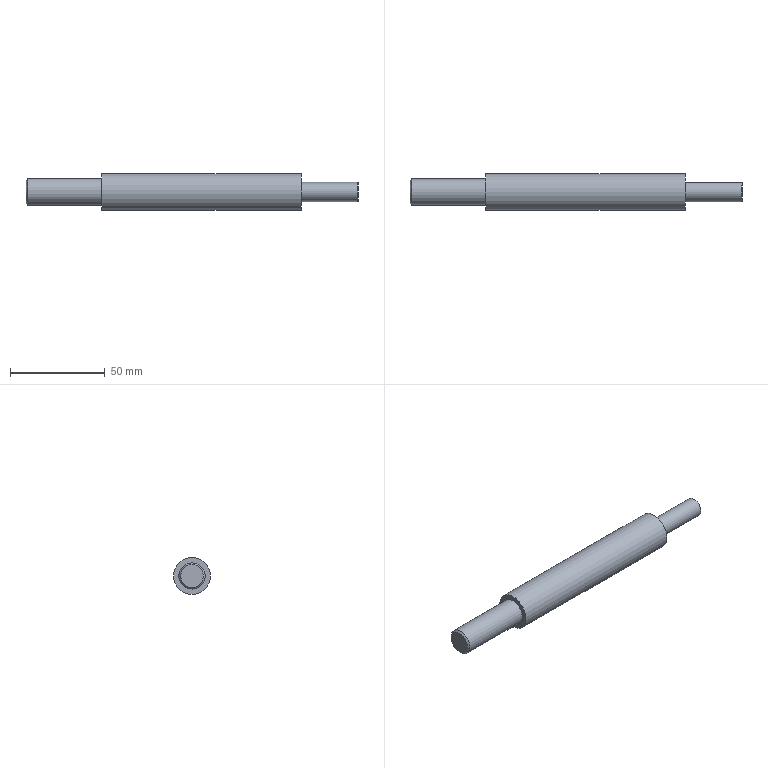Component | NX | THREADED_ROD | 1 solid | 9 faces | box 175 x 19.5 x 19.5 mm | volume 39760 mm3 | plane 4 | cylinder 3 | cone 2 | commonest cylinder face diameters 13.835 x1 19.5 x1 10.106 x1
STEP:
#1=CARTESIAN_POINT('',(0.,0.,0.));
#2=DIRECTION('',(0.,0.,1.));
#3=DIRECTION('',(1.,0.,0.));
#4=AXIS2_PLACEMENT_3D('',#1,#2,#3);
#5=CARTESIAN_POINT('',(-60.,-15.8,139.669));
#6=VERTEX_POINT('',#5);
#7=CARTESIAN_POINT('',(-60.,-15.8,127.669));
#8=VERTEX_POINT('',#7);
#9=CARTESIAN_POINT('',(-60.,-15.8,133.669));
#10=DIRECTION('',(-1.,0.,0.));
#11=DIRECTION('',(0.,0.,1.));
#12=AXIS2_PLACEMENT_3D('',#9,#10,#11);
#13=CIRCLE('',#12,6.);
#14=CARTESIAN_POINT('',(-60.,-15.8,133.669));
#15=DIRECTION('',(-1.,0.,0.));
#16=DIRECTION('',(0.,0.,1.));
#17=AXIS2_PLACEMENT_3D('',#14,#15,#16);
#18=PLANE('',#17);
#19=CARTESIAN_POINT('',(0.,0.));
#20=DIRECTION('',(1.,0.));
#21=AXIS2_PLACEMENT_2D('',#19,#20);
#22=CIRCLE('',#21,6.);
#23=(GEOMETRIC_REPRESENTATION_CONTEXT(2)PARAMETRIC_REPRESENTATION_CONTEXT()REPRESENTATION_CONTEXT('',''));
#24=DEFINITIONAL_REPRESENTATION('',(#22),#23);
#25=PCURVE('',#18,#24);
#26=CARTESIAN_POINT('',(-58.,-15.8,133.669));
#27=DIRECTION('',(1.,0.,0.));
#28=DIRECTION('',(0.,0.,-1.));
#29=AXIS2_PLACEMENT_3D('',#26,#27,#28);
#30=CONICAL_SURFACE('',#29,8.,0.7854);
#31=CARTESIAN_POINT('',(3.142,-2.));
#32=DIRECTION('',(-1.,0.));
#33=VECTOR('',#32,1.);
#34=LINE('',#31,#33);
#35=(GEOMETRIC_REPRESENTATION_CONTEXT(2)PARAMETRIC_REPRESENTATION_CONTEXT()REPRESENTATION_CONTEXT('',''));
#36=DEFINITIONAL_REPRESENTATION('',(#34),#35);
#37=PCURVE('',#30,#36);
#38=SURFACE_CURVE('',#13,(#25,#37),.PCURVE_S1.);
#39=EDGE_CURVE('',#6,#8,#38,.T.);
#40=ORIENTED_EDGE('',*,*,#39,.T.);
#41=CARTESIAN_POINT('',(-60.,-15.8,133.669));
#42=DIRECTION('',(-1.,0.,0.));
#43=DIRECTION('',(0.,0.,1.));
#44=AXIS2_PLACEMENT_3D('',#41,#42,#43);
#45=CIRCLE('',#44,6.);
#46=CARTESIAN_POINT('',(0.,0.));
#47=DIRECTION('',(1.,0.));
#48=AXIS2_PLACEMENT_2D('',#46,#47);
#49=CIRCLE('',#48,6.);
#50=(GEOMETRIC_REPRESENTATION_CONTEXT(2)PARAMETRIC_REPRESENTATION_CONTEXT()REPRESENTATION_CONTEXT('',''));
#51=DEFINITIONAL_REPRESENTATION('',(#49),#50);
#52=PCURVE('',#18,#51);
#53=CARTESIAN_POINT('',(9.425,-2.));
#54=DIRECTION('',(-1.,0.));
#55=VECTOR('',#54,1.);
#56=LINE('',#53,#55);
#57=(GEOMETRIC_REPRESENTATION_CONTEXT(2)PARAMETRIC_REPRESENTATION_CONTEXT()REPRESENTATION_CONTEXT('',''));
#58=DEFINITIONAL_REPRESENTATION('',(#56),#57);
#59=PCURVE('',#30,#58);
#60=SURFACE_CURVE('',#45,(#52,#59),.PCURVE_S1.);
#61=EDGE_CURVE('',#8,#6,#60,.T.);
#62=ORIENTED_EDGE('',*,*,#61,.T.);
#63=EDGE_LOOP('',(#40,#62));
#64=FACE_BOUND('',#63,.T.);
#65=ADVANCED_FACE('',(#64),#18,.T.);
#66=CARTESIAN_POINT('',(-59.083,-15.8,126.752));
#67=VERTEX_POINT('',#66);
#68=CARTESIAN_POINT('',(-59.083,-15.8,133.669));
#69=DIRECTION('',(1.,0.,0.));
#70=DIRECTION('',(0.,0.,-1.));
#71=AXIS2_PLACEMENT_3D('',#68,#69,#70);
#72=CIRCLE('',#71,6.918);
#73=CARTESIAN_POINT('',(-60.,-15.8,133.669));
#74=DIRECTION('',(1.,0.,0.));
#75=DIRECTION('',(0.,0.,-1.));
#76=AXIS2_PLACEMENT_3D('',#73,#74,#75);
#77=CYLINDRICAL_SURFACE('',#76,6.918);
#78=CARTESIAN_POINT('',(0.,0.9175));
#79=DIRECTION('',(1.,0.));
#80=VECTOR('',#79,1.);
#81=LINE('',#78,#80);
#82=(GEOMETRIC_REPRESENTATION_CONTEXT(2)PARAMETRIC_REPRESENTATION_CONTEXT()REPRESENTATION_CONTEXT('',''));
#83=DEFINITIONAL_REPRESENTATION('',(#81),#82);
#84=PCURVE('',#77,#83);
#85=CARTESIAN_POINT('',(0.,-1.083));
#86=DIRECTION('',(1.,0.));
#87=VECTOR('',#86,1.);
#88=LINE('',#85,#87);
#89=(GEOMETRIC_REPRESENTATION_CONTEXT(2)PARAMETRIC_REPRESENTATION_CONTEXT()REPRESENTATION_CONTEXT('',''));
#90=DEFINITIONAL_REPRESENTATION('',(#88),#89);
#91=PCURVE('',#30,#90);
#92=SURFACE_CURVE('',#72,(#84,#91),.PCURVE_S1.);
#93=EDGE_CURVE('',#67,#67,#92,.T.);
#94=ORIENTED_EDGE('',*,*,#93,.T.);
#95=CARTESIAN_POINT('',(-20.,-15.8,126.752));
#96=VERTEX_POINT('',#95);
#97=CARTESIAN_POINT('',(-59.083,-15.8,126.752));
#98=CARTESIAN_POINT('',(-20.,-15.8,126.752));
#99=B_SPLINE_CURVE_WITH_KNOTS('',1,(#97,#98),.UNSPECIFIED.,.F.,.F.,(2,2),(0.9175,40.),.PIECEWISE_BEZIER_KNOTS.);
#100=CARTESIAN_POINT('',(6.283,0.));
#101=DIRECTION('',(0.,1.));
#102=VECTOR('',#101,1.);
#103=LINE('',#100,#102);
#104=(GEOMETRIC_REPRESENTATION_CONTEXT(2)PARAMETRIC_REPRESENTATION_CONTEXT()REPRESENTATION_CONTEXT('',''));
#105=DEFINITIONAL_REPRESENTATION('',(#103),#104);
#106=PCURVE('',#77,#105);
#107=CARTESIAN_POINT('',(0.,0.));
#108=DIRECTION('',(0.,1.));
#109=VECTOR('',#108,1.);
#110=LINE('',#107,#109);
#111=(GEOMETRIC_REPRESENTATION_CONTEXT(2)PARAMETRIC_REPRESENTATION_CONTEXT()REPRESENTATION_CONTEXT('',''));
#112=DEFINITIONAL_REPRESENTATION('',(#110),#111);
#113=PCURVE('',#77,#112);
#114=SEAM_CURVE('',#99,(#106,#113),.PCURVE_S1.);
#115=EDGE_CURVE('',#67,#96,#114,.T.);
#116=ORIENTED_EDGE('',*,*,#115,.T.);
#117=CARTESIAN_POINT('',(-20.,-15.8,140.587));
#118=VERTEX_POINT('',#117);
#119=CARTESIAN_POINT('',(-20.,-15.8,133.669));
#120=DIRECTION('',(-1.,0.,0.));
#121=DIRECTION('',(0.,0.,1.));
#122=AXIS2_PLACEMENT_3D('',#119,#120,#121);
#123=CIRCLE('',#122,6.918);
#124=CARTESIAN_POINT('',(9.425,40.));
#125=DIRECTION('',(-1.,0.));
#126=VECTOR('',#125,1.);
#127=LINE('',#124,#126);
#128=(GEOMETRIC_REPRESENTATION_CONTEXT(2)PARAMETRIC_REPRESENTATION_CONTEXT()REPRESENTATION_CONTEXT('',''));
#129=DEFINITIONAL_REPRESENTATION('',(#127),#128);
#130=PCURVE('',#77,#129);
#131=CARTESIAN_POINT('',(-20.,-15.8,133.669));
#132=DIRECTION('',(-1.,0.,0.));
#133=DIRECTION('',(0.,0.,1.));
#134=AXIS2_PLACEMENT_3D('',#131,#132,#133);
#135=PLANE('',#134);
#136=CARTESIAN_POINT('',(0.,0.));
#137=DIRECTION('',(1.,0.));
#138=AXIS2_PLACEMENT_2D('',#136,#137);
#139=CIRCLE('',#138,6.918);
#140=(GEOMETRIC_REPRESENTATION_CONTEXT(2)PARAMETRIC_REPRESENTATION_CONTEXT()REPRESENTATION_CONTEXT('',''));
#141=DEFINITIONAL_REPRESENTATION('',(#139),#140);
#142=PCURVE('',#135,#141);
#143=SURFACE_CURVE('',#123,(#130,#142),.PCURVE_S1.);
#144=EDGE_CURVE('',#96,#118,#143,.T.);
#145=ORIENTED_EDGE('',*,*,#144,.T.);
#146=CARTESIAN_POINT('',(-20.,-15.8,133.669));
#147=DIRECTION('',(-1.,0.,0.));
#148=DIRECTION('',(0.,0.,1.));
#149=AXIS2_PLACEMENT_3D('',#146,#147,#148);
#150=CIRCLE('',#149,6.918);
#151=CARTESIAN_POINT('',(3.142,40.));
#152=DIRECTION('',(-1.,0.));
#153=VECTOR('',#152,1.);
#154=LINE('',#151,#153);
#155=(GEOMETRIC_REPRESENTATION_CONTEXT(2)PARAMETRIC_REPRESENTATION_CONTEXT()REPRESENTATION_CONTEXT('',''));
#156=DEFINITIONAL_REPRESENTATION('',(#154),#155);
#157=PCURVE('',#77,#156);
#158=CARTESIAN_POINT('',(0.,0.));
#159=DIRECTION('',(1.,0.));
#160=AXIS2_PLACEMENT_2D('',#158,#159);
#161=CIRCLE('',#160,6.918);
#162=(GEOMETRIC_REPRESENTATION_CONTEXT(2)PARAMETRIC_REPRESENTATION_CONTEXT()REPRESENTATION_CONTEXT('',''));
#163=DEFINITIONAL_REPRESENTATION('',(#161),#162);
#164=PCURVE('',#135,#163);
#165=SURFACE_CURVE('',#150,(#157,#164),.PCURVE_S1.);
#166=EDGE_CURVE('',#118,#96,#165,.T.);
#167=ORIENTED_EDGE('',*,*,#166,.T.);
#168=ORIENTED_EDGE('',*,*,#115,.F.);
#169=EDGE_LOOP('',(#94,#116,#145,#167,#168));
#170=FACE_BOUND('',#169,.T.);
#171=ADVANCED_FACE('',(#170),#77,.T.);
#172=CARTESIAN_POINT('',(85.,-15.8,128.616));
#173=VERTEX_POINT('',#172);
#174=CARTESIAN_POINT('',(85.,-15.8,133.669));
#175=DIRECTION('',(1.,0.,0.));
#176=DIRECTION('',(0.,0.,-1.));
#177=AXIS2_PLACEMENT_3D('',#174,#175,#176);
#178=CIRCLE('',#177,5.053);
#179=CARTESIAN_POINT('',(85.,-15.8,133.669));
#180=DIRECTION('',(1.,0.,0.));
#181=DIRECTION('',(0.,0.,-1.));
#182=AXIS2_PLACEMENT_3D('',#179,#180,#181);
#183=PLANE('',#182);
#184=CARTESIAN_POINT('',(0.,0.));
#185=DIRECTION('',(1.,0.));
#186=AXIS2_PLACEMENT_2D('',#184,#185);
#187=CIRCLE('',#186,5.053);
#188=(GEOMETRIC_REPRESENTATION_CONTEXT(2)PARAMETRIC_REPRESENTATION_CONTEXT()REPRESENTATION_CONTEXT('',''));
#189=DEFINITIONAL_REPRESENTATION('',(#187),#188);
#190=PCURVE('',#183,#189);
#191=CARTESIAN_POINT('',(85.,-15.8,133.669));
#192=DIRECTION('',(1.,0.,0.));
#193=DIRECTION('',(0.,0.,-1.));
#194=AXIS2_PLACEMENT_3D('',#191,#192,#193);
#195=CYLINDRICAL_SURFACE('',#194,5.053);
#196=CARTESIAN_POINT('',(0.,0.));
#197=DIRECTION('',(1.,0.));
#198=VECTOR('',#197,1.);
#199=LINE('',#196,#198);
#200=(GEOMETRIC_REPRESENTATION_CONTEXT(2)PARAMETRIC_REPRESENTATION_CONTEXT()REPRESENTATION_CONTEXT('',''));
#201=DEFINITIONAL_REPRESENTATION('',(#199),#200);
#202=PCURVE('',#195,#201);
#203=SURFACE_CURVE('',#178,(#190,#202),.PCURVE_S1.);
#204=EDGE_CURVE('',#173,#173,#203,.T.);
#205=ORIENTED_EDGE('',*,*,#204,.F.);
#206=EDGE_LOOP('',(#205));
#207=FACE_BOUND('',#206,.T.);
#208=CARTESIAN_POINT('',(85.,-15.8,123.919));
#209=VERTEX_POINT('',#208);
#210=CARTESIAN_POINT('',(85.,-15.8,133.669));
#211=DIRECTION('',(-1.,0.,0.));
#212=DIRECTION('',(0.,0.,-1.));
#213=AXIS2_PLACEMENT_3D('',#210,#211,#212);
#214=CIRCLE('',#213,9.75);
#215=CARTESIAN_POINT('',(9.75,0.));
#216=CARTESIAN_POINT('',(9.75,-16.887));
#217=CARTESIAN_POINT('',(-4.875,-8.444));
#218=CARTESIAN_POINT('',(-19.5,-0.));
#219=CARTESIAN_POINT('',(-4.875,8.444));
#220=CARTESIAN_POINT('',(9.75,16.887));
#221=CARTESIAN_POINT('',(9.75,0.));
#222=(BOUNDED_CURVE()B_SPLINE_CURVE(2,(#215,#216,#217,#218,#219,#220,#221),.UNSPECIFIED.,.T.,.F.)B_SPLINE_CURVE_WITH_KNOTS((1,2,2,2,2,1),(-2.094,0.,2.094,4.189,6.283,8.378),.UNSPECIFIED.)CURVE()GEOMETRIC_REPRESENTATION_ITEM()RATIONAL_B_SPLINE_CURVE((1.,0.5,1.,0.5,1.,0.5,1.))REPRESENTATION_ITEM(''));
#223=(GEOMETRIC_REPRESENTATION_CONTEXT(2)PARAMETRIC_REPRESENTATION_CONTEXT()REPRESENTATION_CONTEXT('',''));
#224=DEFINITIONAL_REPRESENTATION('',(#222),#223);
#225=PCURVE('',#183,#224);
#226=CARTESIAN_POINT('',(-20.,-15.8,133.669));
#227=DIRECTION('',(1.,0.,0.));
#228=DIRECTION('',(0.,0.,-1.));
#229=AXIS2_PLACEMENT_3D('',#226,#227,#228);
#230=CYLINDRICAL_SURFACE('',#229,9.75);
#231=CARTESIAN_POINT('',(6.283,105.));
#232=DIRECTION('',(-1.,0.));
#233=VECTOR('',#232,1.);
#234=LINE('',#231,#233);
#235=(GEOMETRIC_REPRESENTATION_CONTEXT(2)PARAMETRIC_REPRESENTATION_CONTEXT()REPRESENTATION_CONTEXT('',''));
#236=DEFINITIONAL_REPRESENTATION('',(#234),#235);
#237=PCURVE('',#230,#236);
#238=SURFACE_CURVE('',#214,(#225,#237),.PCURVE_S1.);
#239=EDGE_CURVE('',#209,#209,#238,.T.);
#240=ORIENTED_EDGE('',*,*,#239,.F.);
#241=EDGE_LOOP('',(#240));
#242=FACE_BOUND('',#241,.T.);
#243=ADVANCED_FACE('',(#207,#242),#183,.T.);
#244=ORIENTED_EDGE('',*,*,#166,.F.);
#245=ORIENTED_EDGE('',*,*,#144,.F.);
#246=EDGE_LOOP('',(#244,#245));
#247=FACE_BOUND('',#246,.T.);
#248=CARTESIAN_POINT('',(-20.,-15.8,123.919));
#249=VERTEX_POINT('',#248);
#250=CARTESIAN_POINT('',(-20.,-15.8,133.669));
#251=DIRECTION('',(1.,0.,0.));
#252=DIRECTION('',(0.,0.,-1.));
#253=AXIS2_PLACEMENT_3D('',#250,#251,#252);
#254=CIRCLE('',#253,9.75);
#255=CARTESIAN_POINT('',(-9.75,0.));
#256=CARTESIAN_POINT('',(-9.75,16.887));
#257=CARTESIAN_POINT('',(4.875,8.444));
#258=CARTESIAN_POINT('',(19.5,0.));
#259=CARTESIAN_POINT('',(4.875,-8.444));
#260=CARTESIAN_POINT('',(-9.75,-16.887));
#261=CARTESIAN_POINT('',(-9.75,0.));
#262=(BOUNDED_CURVE()B_SPLINE_CURVE(2,(#255,#256,#257,#258,#259,#260,#261),.UNSPECIFIED.,.T.,.F.)B_SPLINE_CURVE_WITH_KNOTS((1,2,2,2,2,1),(-2.094,0.,2.094,4.189,6.283,8.378),.UNSPECIFIED.)CURVE()GEOMETRIC_REPRESENTATION_ITEM()RATIONAL_B_SPLINE_CURVE((1.,0.5,1.,0.5,1.,0.5,1.))REPRESENTATION_ITEM(''));
#263=(GEOMETRIC_REPRESENTATION_CONTEXT(2)PARAMETRIC_REPRESENTATION_CONTEXT()REPRESENTATION_CONTEXT('',''));
#264=DEFINITIONAL_REPRESENTATION('',(#262),#263);
#265=PCURVE('',#135,#264);
#266=CARTESIAN_POINT('',(0.,0.));
#267=DIRECTION('',(1.,0.));
#268=VECTOR('',#267,1.);
#269=LINE('',#266,#268);
#270=(GEOMETRIC_REPRESENTATION_CONTEXT(2)PARAMETRIC_REPRESENTATION_CONTEXT()REPRESENTATION_CONTEXT('',''));
#271=DEFINITIONAL_REPRESENTATION('',(#269),#270);
#272=PCURVE('',#230,#271);
#273=SURFACE_CURVE('',#254,(#265,#272),.PCURVE_S1.);
#274=EDGE_CURVE('',#249,#249,#273,.T.);
#275=ORIENTED_EDGE('',*,*,#274,.F.);
#276=EDGE_LOOP('',(#275));
#277=FACE_BOUND('',#276,.T.);
#278=ADVANCED_FACE('',(#247,#277),#135,.T.);
#279=ORIENTED_EDGE('',*,*,#239,.T.);
#280=CARTESIAN_POINT('',(-20.,-15.8,123.919));
#281=CARTESIAN_POINT('',(85.,-15.8,123.919));
#282=B_SPLINE_CURVE_WITH_KNOTS('',1,(#280,#281),.UNSPECIFIED.,.F.,.F.,(2,2),(0.,105.),.PIECEWISE_BEZIER_KNOTS.);
#283=CARTESIAN_POINT('',(0.,0.));
#284=DIRECTION('',(0.,1.));
#285=VECTOR('',#284,1.);
#286=LINE('',#283,#285);
#287=(GEOMETRIC_REPRESENTATION_CONTEXT(2)PARAMETRIC_REPRESENTATION_CONTEXT()REPRESENTATION_CONTEXT('',''));
#288=DEFINITIONAL_REPRESENTATION('',(#286),#287);
#289=PCURVE('',#230,#288);
#290=CARTESIAN_POINT('',(6.283,0.));
#291=DIRECTION('',(0.,1.));
#292=VECTOR('',#291,1.);
#293=LINE('',#290,#292);
#294=(GEOMETRIC_REPRESENTATION_CONTEXT(2)PARAMETRIC_REPRESENTATION_CONTEXT()REPRESENTATION_CONTEXT('',''));
#295=DEFINITIONAL_REPRESENTATION('',(#293),#294);
#296=PCURVE('',#230,#295);
#297=SEAM_CURVE('',#282,(#289,#296),.PCURVE_S1.);
#298=EDGE_CURVE('',#249,#209,#297,.T.);
#299=ORIENTED_EDGE('',*,*,#298,.F.);
#300=ORIENTED_EDGE('',*,*,#274,.T.);
#301=ORIENTED_EDGE('',*,*,#298,.T.);
#302=EDGE_LOOP('',(#279,#299,#300,#301));
#303=FACE_BOUND('',#302,.T.);
#304=ADVANCED_FACE('',(#303),#230,.T.);
#305=CARTESIAN_POINT('',(115.,-15.8,128.669));
#306=VERTEX_POINT('',#305);
#307=CARTESIAN_POINT('',(115.,-15.8,133.669));
#308=DIRECTION('',(1.,0.,0.));
#309=DIRECTION('',(0.,0.,-1.));
#310=AXIS2_PLACEMENT_3D('',#307,#308,#309);
#311=CIRCLE('',#310,5.);
#312=CARTESIAN_POINT('',(115.,-15.8,133.669));
#313=DIRECTION('',(1.,0.,0.));
#314=DIRECTION('',(0.,0.,-1.));
#315=AXIS2_PLACEMENT_3D('',#312,#313,#314);
#316=PLANE('',#315);
#317=CARTESIAN_POINT('',(0.,0.));
#318=DIRECTION('',(1.,0.));
#319=AXIS2_PLACEMENT_2D('',#317,#318);
#320=CIRCLE('',#319,5.);
#321=(GEOMETRIC_REPRESENTATION_CONTEXT(2)PARAMETRIC_REPRESENTATION_CONTEXT()REPRESENTATION_CONTEXT('',''));
#322=DEFINITIONAL_REPRESENTATION('',(#320),#321);
#323=PCURVE('',#316,#322);
#324=CARTESIAN_POINT('',(114.,-15.8,133.669));
#325=DIRECTION('',(-1.,0.,0.));
#326=DIRECTION('',(0.,0.,1.));
#327=AXIS2_PLACEMENT_3D('',#324,#325,#326);
#328=CONICAL_SURFACE('',#327,6.,0.7854);
#329=CARTESIAN_POINT('',(9.425,-1.));
#330=DIRECTION('',(-1.,0.));
#331=VECTOR('',#330,1.);
#332=LINE('',#329,#331);
#333=(GEOMETRIC_REPRESENTATION_CONTEXT(2)PARAMETRIC_REPRESENTATION_CONTEXT()REPRESENTATION_CONTEXT('',''));
#334=DEFINITIONAL_REPRESENTATION('',(#332),#333);
#335=PCURVE('',#328,#334);
#336=SURFACE_CURVE('',#311,(#323,#335),.PCURVE_S1.);
#337=EDGE_CURVE('',#306,#306,#336,.T.);
#338=ORIENTED_EDGE('',*,*,#337,.T.);
#339=EDGE_LOOP('',(#338));
#340=FACE_BOUND('',#339,.T.);
#341=ADVANCED_FACE('',(#340),#316,.T.);
#342=CARTESIAN_POINT('',(114.947,-15.8,138.722));
#343=VERTEX_POINT('',#342);
#344=CARTESIAN_POINT('',(114.947,-15.8,128.616));
#345=VERTEX_POINT('',#344);
#346=CARTESIAN_POINT('',(114.947,-15.8,133.669));
#347=DIRECTION('',(-1.,0.,0.));
#348=DIRECTION('',(0.,0.,1.));
#349=AXIS2_PLACEMENT_3D('',#346,#347,#348);
#350=CIRCLE('',#349,5.053);
#351=CARTESIAN_POINT('',(3.142,29.947));
#352=DIRECTION('',(-1.,0.));
#353=VECTOR('',#352,1.);
#354=LINE('',#351,#353);
#355=(GEOMETRIC_REPRESENTATION_CONTEXT(2)PARAMETRIC_REPRESENTATION_CONTEXT()REPRESENTATION_CONTEXT('',''));
#356=DEFINITIONAL_REPRESENTATION('',(#354),#355);
#357=PCURVE('',#195,#356);
#358=CARTESIAN_POINT('',(6.283,-0.947));
#359=DIRECTION('',(1.,0.));
#360=VECTOR('',#359,1.);
#361=LINE('',#358,#360);
#362=(GEOMETRIC_REPRESENTATION_CONTEXT(2)PARAMETRIC_REPRESENTATION_CONTEXT()REPRESENTATION_CONTEXT('',''));
#363=DEFINITIONAL_REPRESENTATION('',(#361),#362);
#364=PCURVE('',#328,#363);
#365=SURFACE_CURVE('',#350,(#357,#364),.PCURVE_S1.);
#366=EDGE_CURVE('',#343,#345,#365,.T.);
#367=ORIENTED_EDGE('',*,*,#366,.T.);
#368=CARTESIAN_POINT('',(85.,-15.8,128.616));
#369=CARTESIAN_POINT('',(114.947,-15.8,128.616));
#370=B_SPLINE_CURVE_WITH_KNOTS('',1,(#368,#369),.UNSPECIFIED.,.F.,.F.,(2,2),(0.,29.947),.PIECEWISE_BEZIER_KNOTS.);
#371=CARTESIAN_POINT('',(0.,0.));
#372=DIRECTION('',(0.,1.));
#373=VECTOR('',#372,1.);
#374=LINE('',#371,#373);
#375=(GEOMETRIC_REPRESENTATION_CONTEXT(2)PARAMETRIC_REPRESENTATION_CONTEXT()REPRESENTATION_CONTEXT('',''));
#376=DEFINITIONAL_REPRESENTATION('',(#374),#375);
#377=PCURVE('',#195,#376);
#378=CARTESIAN_POINT('',(6.283,0.));
#379=DIRECTION('',(0.,1.));
#380=VECTOR('',#379,1.);
#381=LINE('',#378,#380);
#382=(GEOMETRIC_REPRESENTATION_CONTEXT(2)PARAMETRIC_REPRESENTATION_CONTEXT()REPRESENTATION_CONTEXT('',''));
#383=DEFINITIONAL_REPRESENTATION('',(#381),#382);
#384=PCURVE('',#195,#383);
#385=SEAM_CURVE('',#370,(#377,#384),.PCURVE_S1.);
#386=EDGE_CURVE('',#173,#345,#385,.T.);
#387=ORIENTED_EDGE('',*,*,#386,.F.);
#388=ORIENTED_EDGE('',*,*,#204,.T.);
#389=ORIENTED_EDGE('',*,*,#386,.T.);
#390=CARTESIAN_POINT('',(114.947,-15.8,133.669));
#391=DIRECTION('',(-1.,0.,0.));
#392=DIRECTION('',(0.,0.,1.));
#393=AXIS2_PLACEMENT_3D('',#390,#391,#392);
#394=CIRCLE('',#393,5.053);
#395=CARTESIAN_POINT('',(9.425,29.947));
#396=DIRECTION('',(-1.,0.));
#397=VECTOR('',#396,1.);
#398=LINE('',#395,#397);
#399=(GEOMETRIC_REPRESENTATION_CONTEXT(2)PARAMETRIC_REPRESENTATION_CONTEXT()REPRESENTATION_CONTEXT('',''));
#400=DEFINITIONAL_REPRESENTATION('',(#398),#399);
#401=PCURVE('',#195,#400);
#402=CARTESIAN_POINT('',(0.,-0.947));
#403=DIRECTION('',(1.,0.));
#404=VECTOR('',#403,1.);
#405=LINE('',#402,#404);
#406=(GEOMETRIC_REPRESENTATION_CONTEXT(2)PARAMETRIC_REPRESENTATION_CONTEXT()REPRESENTATION_CONTEXT('',''));
#407=DEFINITIONAL_REPRESENTATION('',(#405),#406);
#408=PCURVE('',#328,#407);
#409=SURFACE_CURVE('',#394,(#401,#408),.PCURVE_S1.);
#410=EDGE_CURVE('',#345,#343,#409,.T.);
#411=ORIENTED_EDGE('',*,*,#410,.T.);
#412=EDGE_LOOP('',(#367,#387,#388,#389,#411));
#413=FACE_BOUND('',#412,.T.);
#414=ADVANCED_FACE('',(#413),#195,.T.);
#415=ORIENTED_EDGE('',*,*,#337,.F.);
#416=CARTESIAN_POINT('',(115.,-15.8,128.669));
#417=CARTESIAN_POINT('',(114.947,-15.8,128.616));
#418=B_SPLINE_CURVE_WITH_KNOTS('',1,(#416,#417),.UNSPECIFIED.,.F.,.F.,(2,2),(-1.414,-1.339),.PIECEWISE_BEZIER_KNOTS.);
#419=CARTESIAN_POINT('',(9.425,0.));
#420=DIRECTION('',(0.,1.));
#421=VECTOR('',#420,1.);
#422=LINE('',#419,#421);
#423=(GEOMETRIC_REPRESENTATION_CONTEXT(2)PARAMETRIC_REPRESENTATION_CONTEXT()REPRESENTATION_CONTEXT('',''));
#424=DEFINITIONAL_REPRESENTATION('',(#422),#423);
#425=PCURVE('',#328,#424);
#426=CARTESIAN_POINT('',(3.142,0.));
#427=DIRECTION('',(0.,1.));
#428=VECTOR('',#427,1.);
#429=LINE('',#426,#428);
#430=(GEOMETRIC_REPRESENTATION_CONTEXT(2)PARAMETRIC_REPRESENTATION_CONTEXT()REPRESENTATION_CONTEXT('',''));
#431=DEFINITIONAL_REPRESENTATION('',(#429),#430);
#432=PCURVE('',#328,#431);
#433=SEAM_CURVE('',#418,(#425,#432),.PCURVE_S1.);
#434=EDGE_CURVE('',#306,#345,#433,.T.);
#435=ORIENTED_EDGE('',*,*,#434,.T.);
#436=ORIENTED_EDGE('',*,*,#366,.F.);
#437=ORIENTED_EDGE('',*,*,#410,.F.);
#438=ORIENTED_EDGE('',*,*,#434,.F.);
#439=EDGE_LOOP('',(#415,#435,#436,#437,#438));
#440=FACE_BOUND('',#439,.T.);
#441=ADVANCED_FACE('',(#440),#328,.T.);
#442=ORIENTED_EDGE('',*,*,#61,.F.);
#443=CARTESIAN_POINT('',(-60.,-15.8,127.669));
#444=CARTESIAN_POINT('',(-59.083,-15.8,126.752));
#445=B_SPLINE_CURVE_WITH_KNOTS('',1,(#443,#444),.UNSPECIFIED.,.F.,.F.,(2,2),(-2.828,-1.531),.PIECEWISE_BEZIER_KNOTS.);
#446=CARTESIAN_POINT('',(6.283,0.));
#447=DIRECTION('',(0.,1.));
#448=VECTOR('',#447,1.);
#449=LINE('',#446,#448);
#450=(GEOMETRIC_REPRESENTATION_CONTEXT(2)PARAMETRIC_REPRESENTATION_CONTEXT()REPRESENTATION_CONTEXT('',''));
#451=DEFINITIONAL_REPRESENTATION('',(#449),#450);
#452=PCURVE('',#30,#451);
#453=CARTESIAN_POINT('',(0.,0.));
#454=DIRECTION('',(0.,1.));
#455=VECTOR('',#454,1.);
#456=LINE('',#453,#455);
#457=(GEOMETRIC_REPRESENTATION_CONTEXT(2)PARAMETRIC_REPRESENTATION_CONTEXT()REPRESENTATION_CONTEXT('',''));
#458=DEFINITIONAL_REPRESENTATION('',(#456),#457);
#459=PCURVE('',#30,#458);
#460=SEAM_CURVE('',#445,(#452,#459),.PCURVE_S1.);
#461=EDGE_CURVE('',#8,#67,#460,.T.);
#462=ORIENTED_EDGE('',*,*,#461,.T.);
#463=ORIENTED_EDGE('',*,*,#93,.F.);
#464=ORIENTED_EDGE('',*,*,#461,.F.);
#465=ORIENTED_EDGE('',*,*,#39,.F.);
#466=EDGE_LOOP('',(#442,#462,#463,#464,#465));
#467=FACE_BOUND('',#466,.T.);
#468=ADVANCED_FACE('',(#467),#30,.T.);
#469=CLOSED_SHELL('',(#65,#171,#243,#278,#304,#341,#414,#441,#468));
#470=MANIFOLD_SOLID_BREP('',#469);
#471=(LENGTH_UNIT()NAMED_UNIT(*)SI_UNIT(.MILLI.,.METRE.));
#472=UNCERTAINTY_MEASURE_WITH_UNIT(LENGTH_MEASURE(0.000005),#471,'','');
#473=(NAMED_UNIT(*)PLANE_ANGLE_UNIT()SI_UNIT($,.RADIAN.));
#474=(NAMED_UNIT(*)SI_UNIT($,.STERADIAN.)SOLID_ANGLE_UNIT());
#475=(GEOMETRIC_REPRESENTATION_CONTEXT(3)GLOBAL_UNCERTAINTY_ASSIGNED_CONTEXT((#472))GLOBAL_UNIT_ASSIGNED_CONTEXT((#471,#473,#474))REPRESENTATION_CONTEXT('',''));
#476=ADVANCED_BREP_SHAPE_REPRESENTATION('',(#4,#470),#475);